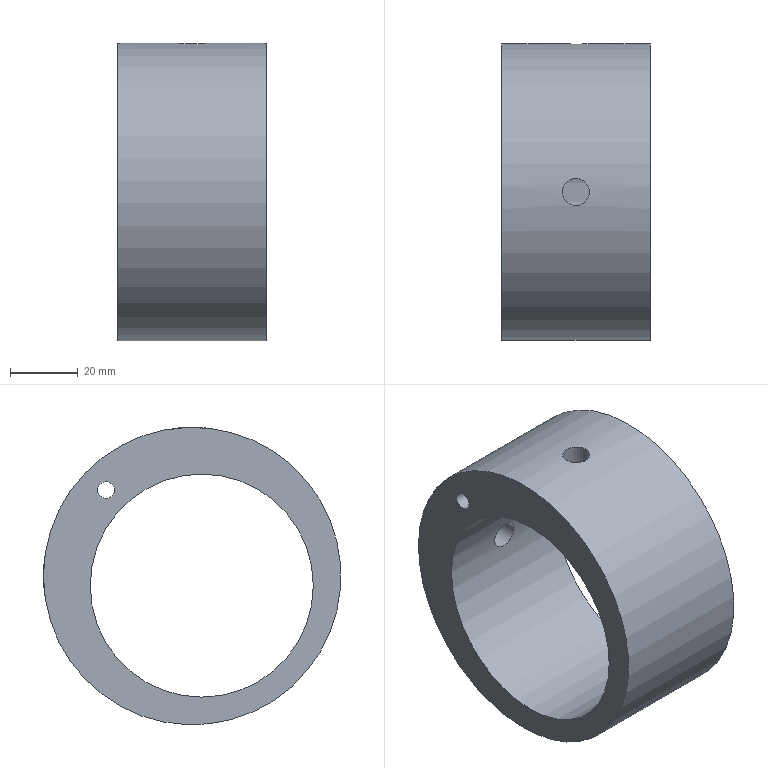Component | NX | ECCENTRIC_SLEEVE | 1 solid | 7 faces | volume 114813 mm3 | cylinder 5 | plane 2 | commonest cylinder face diameters 8 x2 88 x1 5 x1 66 x1